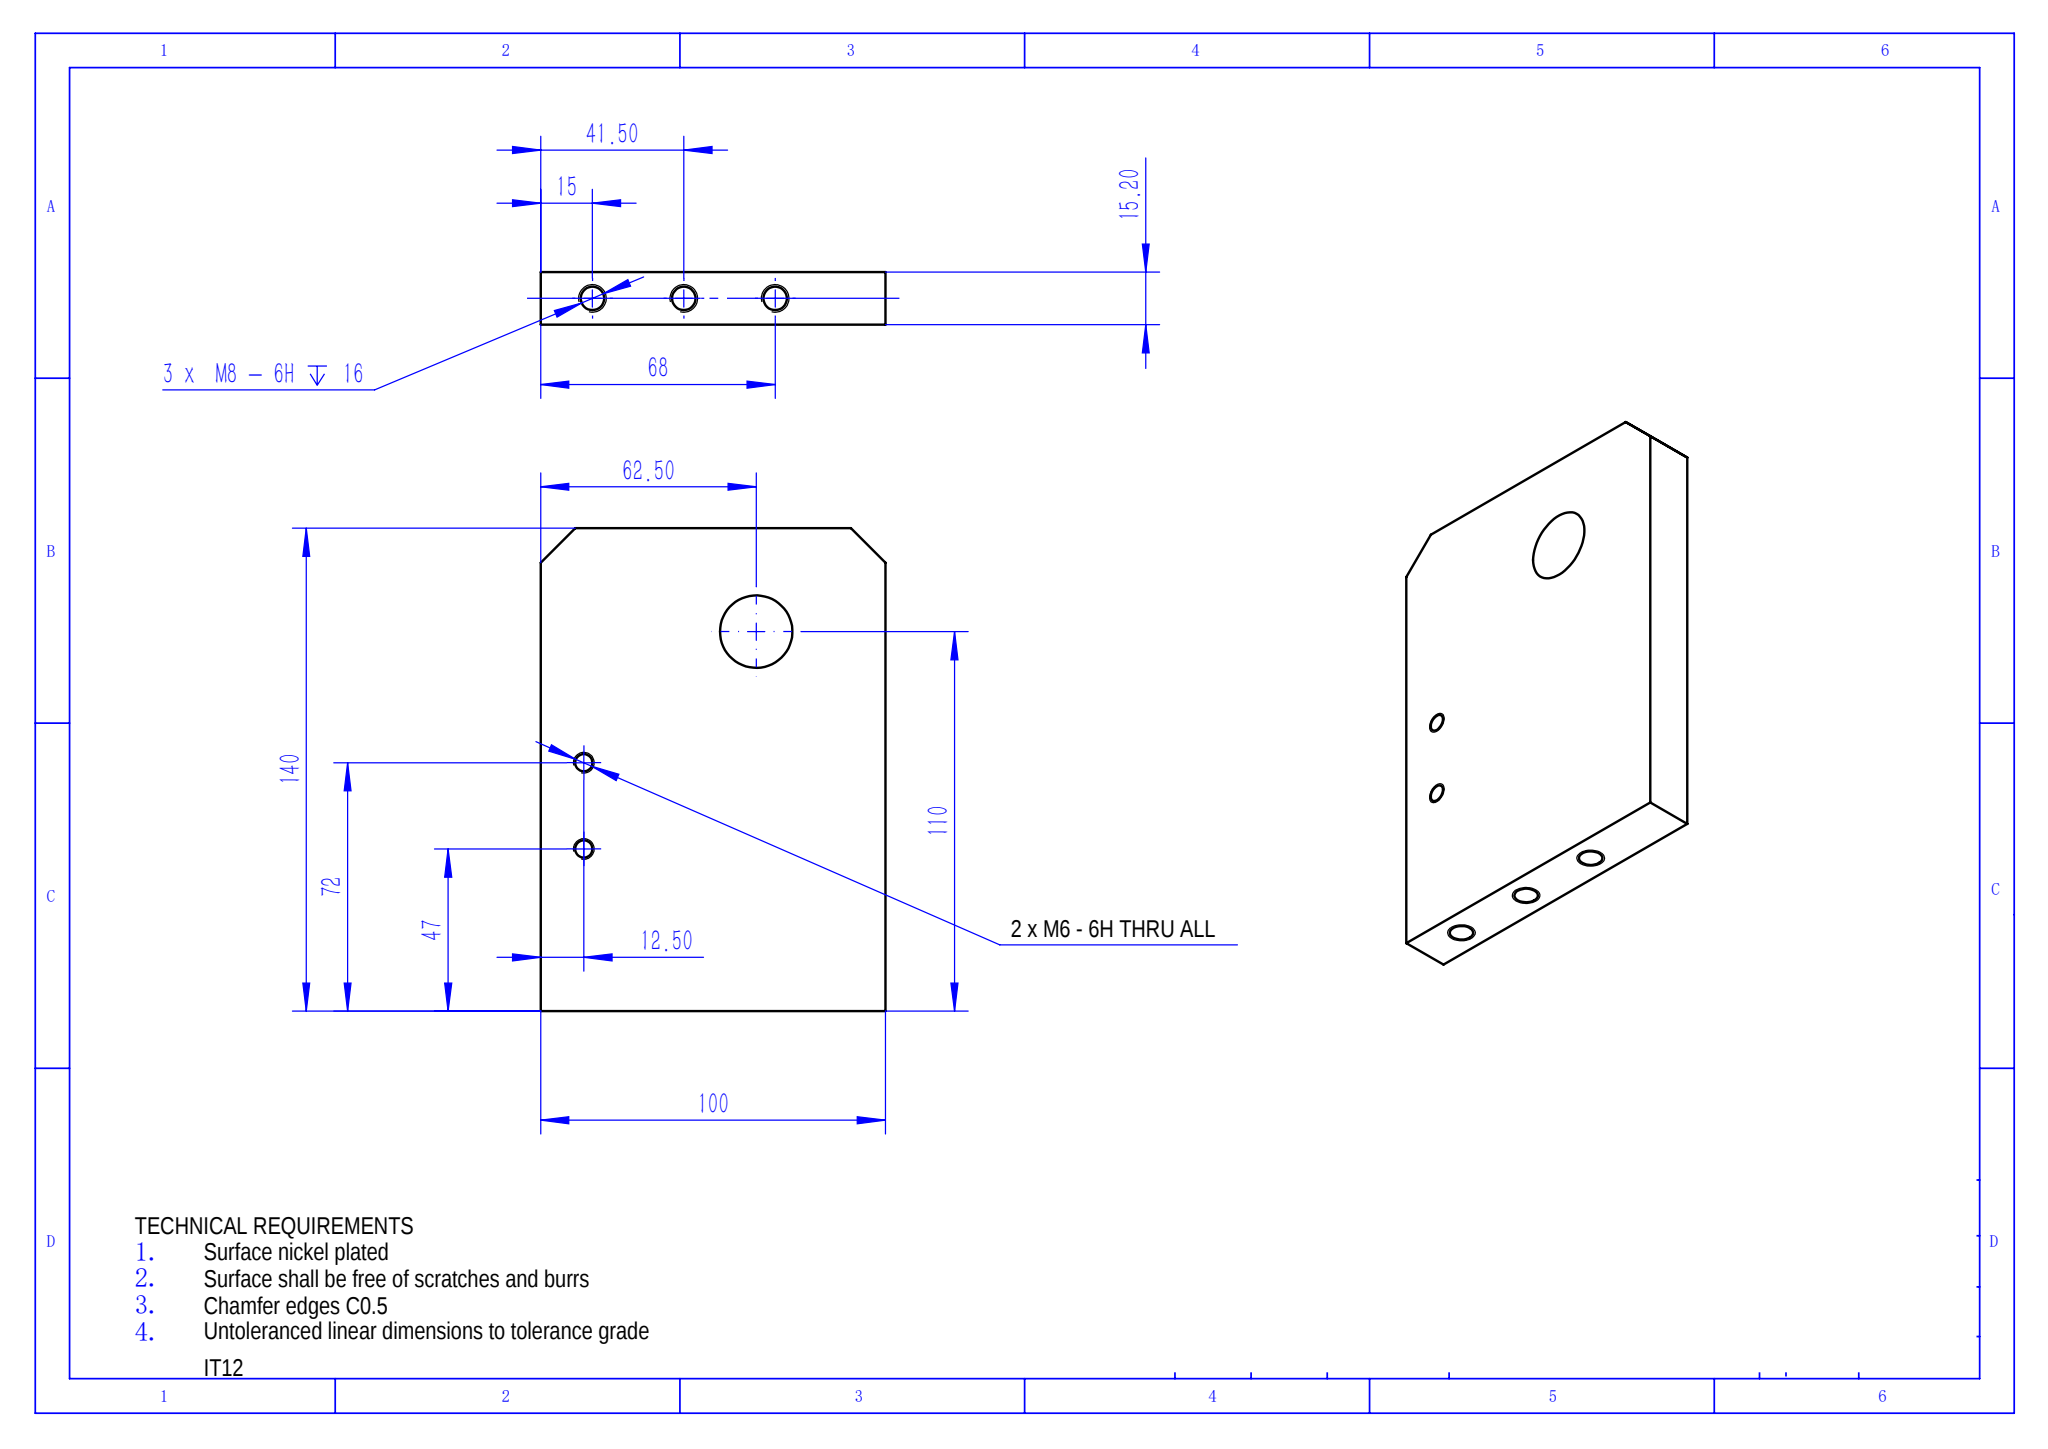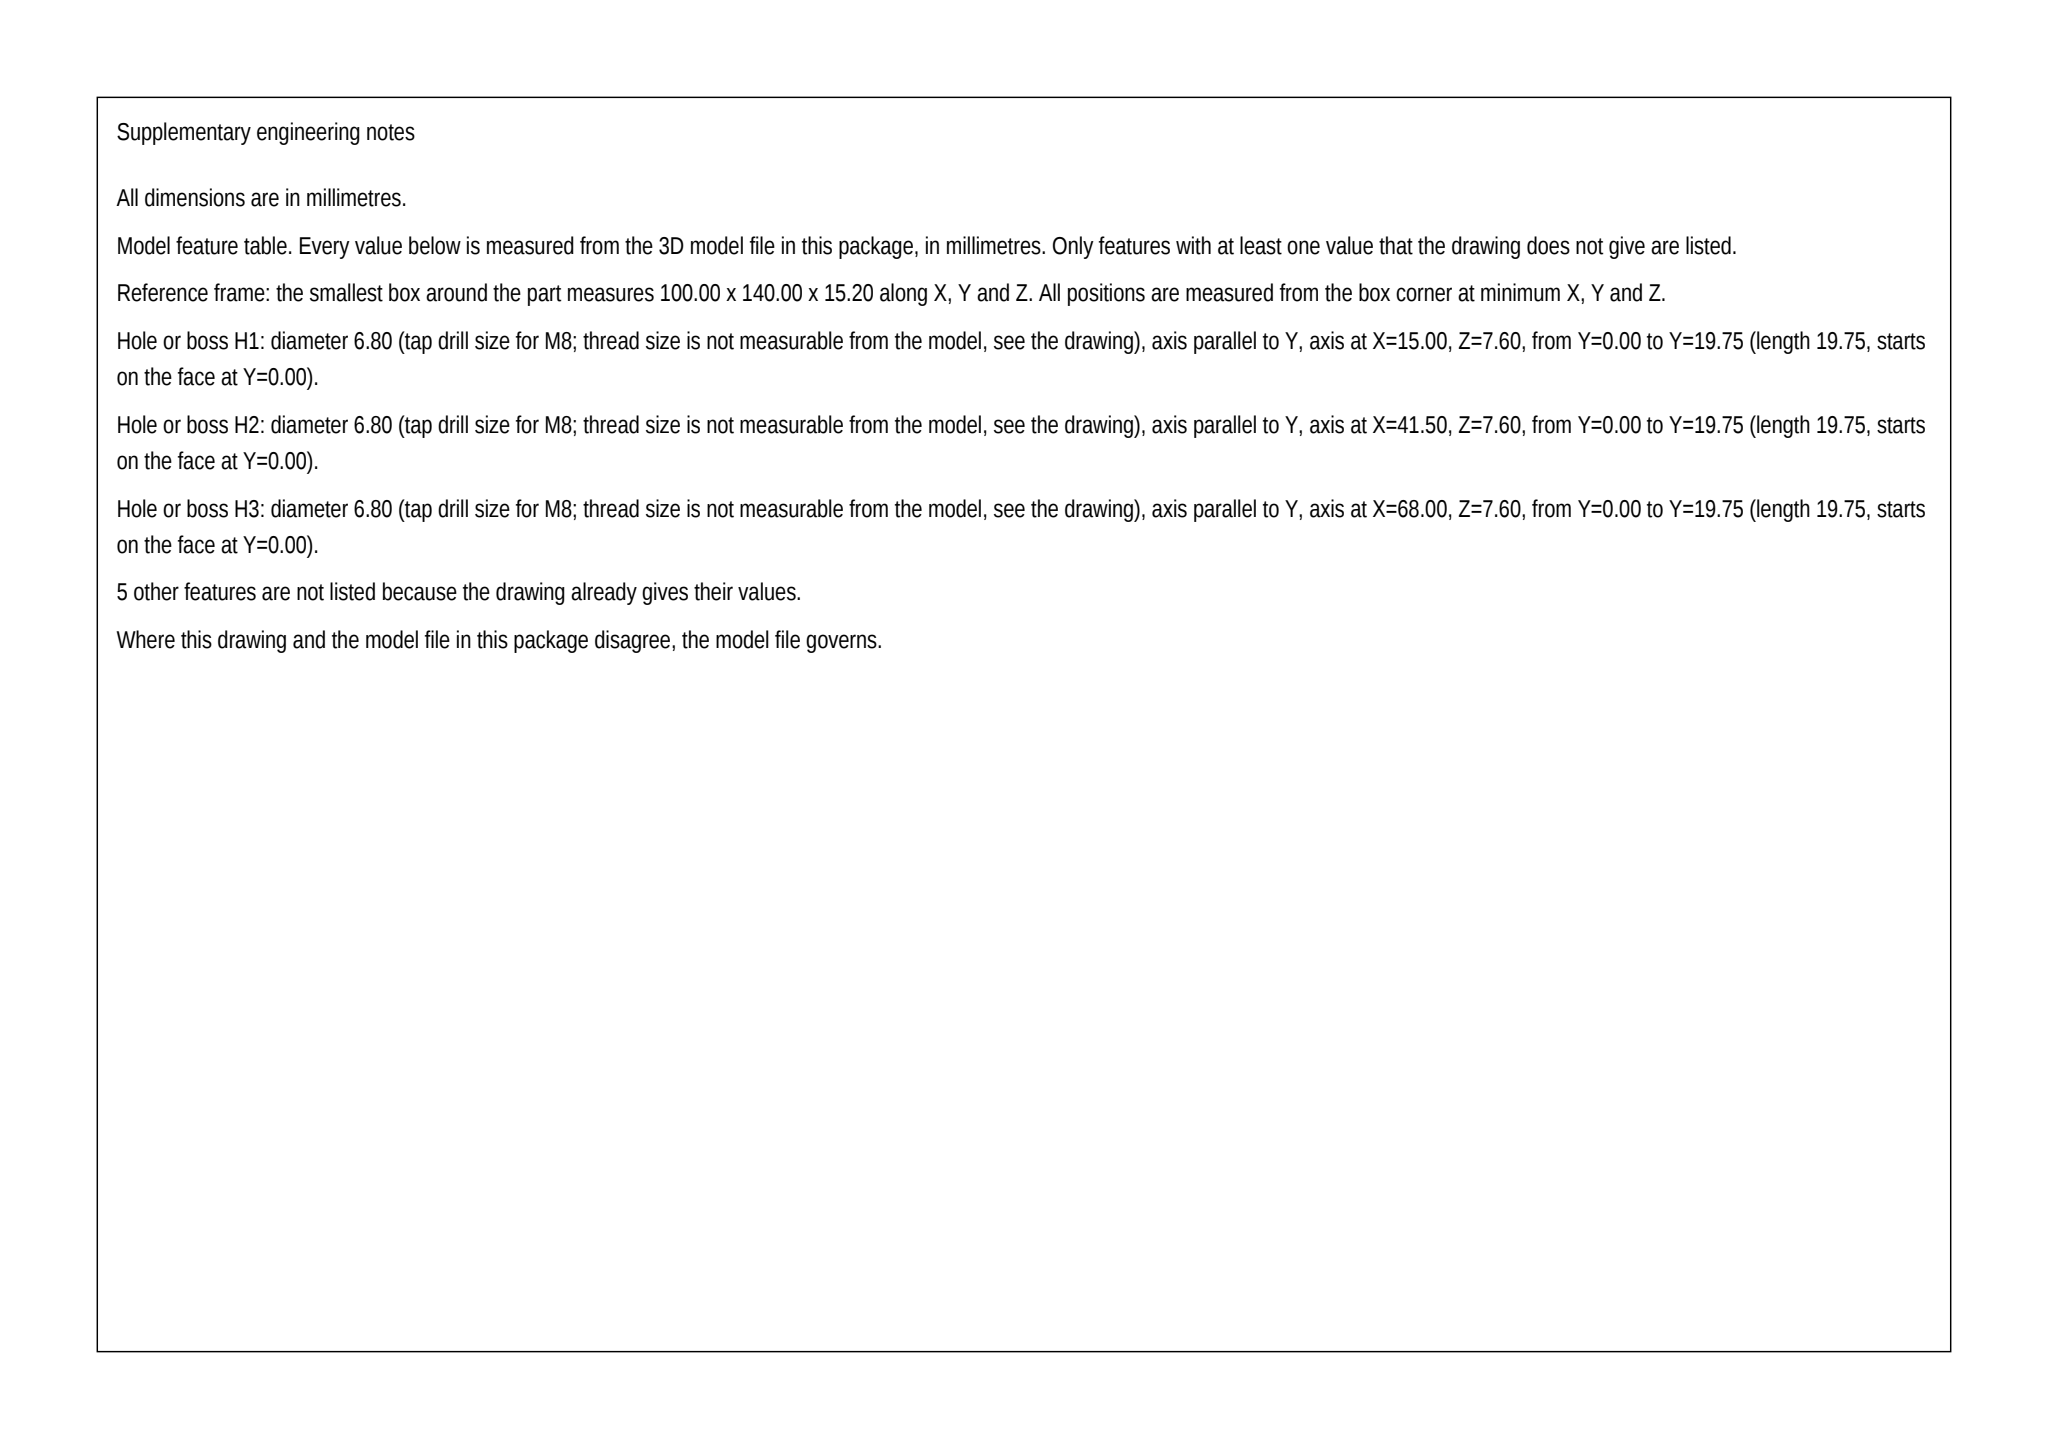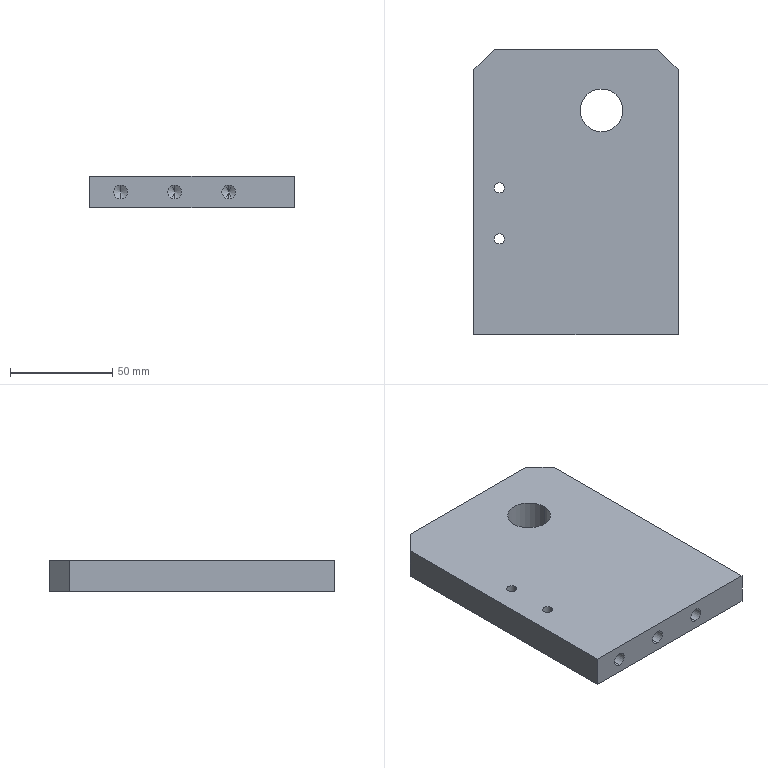Part | SolidWorks | mm | 1 solid | 26 faces | box 100 x 140 x 15.2 mm | volume 203192 mm3 | cylinder 12 | plane 8 | cone 6 | commonest cylinder face diameters 6.8 x6 5 x4 21 x2
Drawing notes:
FRONT VIEW: 2X C10 CHAMFER AT TOP CORNERS | from the solid: 100x140x15.2 plate, two cut corners on top edge of 140 face; chamfer legs 10
1X Ø21 THRU, 62.50 FROM LH EDGE, 110 FROM BOTTOM EDGE | from the solid: cylinder dia 21.0, axis z, pos (62.5,110.0), length 15.2 = full thickness
build123d program:
from build123d import *

# Parameters (mm, degrees)
SKETCH1_W             = 100
SKETCH1_H             = 140
BOSS_EXTRUDE1_DEPTH   = 15.2
SKETCH4_R             = 10.5
CUT_EXTRUDE1_DEPTH    = 173.717
CHAMFER1_SIZE         = 10
M8_TAPPED_HOLE2_D     = 6.8
M8_TAPPED_HOLE2_DEPTH = 19.75
M8_TAPPED_HOLE2_TIP   = 2.043
M6_TAPPED_HOLE2_D     = 5


with BuildPart() as part:
    # Sketch1 → Boss-Extrude1 (new body)
    with BuildSketch(Plane.XY):
        with Locations((50, 70)):
            Rectangle(SKETCH1_W, SKETCH1_H)
    extrude(amount=BOSS_EXTRUDE1_DEPTH)

    # Sketch4 → Cut-Extrude1 (cut, through all)
    with BuildSketch(Plane(origin=(0, 0, 0), x_dir=(-1, 0, 0), z_dir=(0, 0, -1))):
        with Locations((-62.5, 110)):
            Circle(SKETCH4_R)
    extrude(amount=-CUT_EXTRUDE1_DEPTH, mode=Mode.SUBTRACT)

    # Chamfer1
    chamfer1_edges = [part.edges().sort_by_distance(p)[0] for p in [
        (0, 140, 7.6),
        (100, 140, 7.6),
    ]]
    chamfer(chamfer1_edges, length=CHAMFER1_SIZE)

    # M8 Tapped Hole2
    with Locations(Plane(origin=(0, 0, 0), x_dir=(-1, 0, 0), z_dir=(0, -1, 0))):
        with Locations((-15, -7.6), (-41.5, -7.6), (-68, -7.6)):
            Hole(M8_TAPPED_HOLE2_D / 2, depth=M8_TAPPED_HOLE2_DEPTH)
            with Locations((0, 0, -(M8_TAPPED_HOLE2_DEPTH + M8_TAPPED_HOLE2_TIP / 2))):  # 118° drill point
                Cone(0, M8_TAPPED_HOLE2_D / 2, M8_TAPPED_HOLE2_TIP, mode=Mode.SUBTRACT)

    # M6 Tapped Hole2 (through all)
    with Locations(Plane.XY.offset(15.2)):
        with Locations((12.5, 72), (12.5, 47)):
            Hole(M6_TAPPED_HOLE2_D / 2)


solid = part.part
STEP:
#1=CARTESIAN_POINT('',(10.,72.,0.));
#2=VERTEX_POINT('',#1);
#3=CARTESIAN_POINT('',(15.,72.,0.));
#4=VERTEX_POINT('',#3);
#5=CARTESIAN_POINT('',(12.5,72.,0.));
#6=DIRECTION('',(0.,0.,1.));
#7=DIRECTION('',(1.,0.,0.));
#8=AXIS2_PLACEMENT_3D('',#5,#6,#7);
#9=CIRCLE('',#8,2.5);
#10=EDGE_CURVE('',#2,#4,#9,.T.);
#11=ORIENTED_EDGE('',*,*,#10,.F.);
#12=CARTESIAN_POINT('',(10.,72.,15.2));
#13=VERTEX_POINT('',#12);
#14=CARTESIAN_POINT('',(10.,72.,15.2));
#15=DIRECTION('',(0.,0.,1.));
#16=VECTOR('',#15,1000.);
#17=LINE('',#14,#16);
#18=EDGE_CURVE('',#2,#13,#17,.T.);
#19=ORIENTED_EDGE('',*,*,#18,.T.);
#20=CARTESIAN_POINT('',(15.,72.,15.2));
#21=VERTEX_POINT('',#20);
#22=CARTESIAN_POINT('',(12.5,72.,15.2));
#23=DIRECTION('',(0.,0.,1.));
#24=DIRECTION('',(1.,0.,0.));
#25=AXIS2_PLACEMENT_3D('',#22,#23,#24);
#26=CIRCLE('',#25,2.5);
#27=EDGE_CURVE('',#13,#21,#26,.T.);
#28=ORIENTED_EDGE('',*,*,#27,.T.);
#29=CARTESIAN_POINT('',(15.,72.,15.2));
#30=DIRECTION('',(0.,0.,1.));
#31=VECTOR('',#30,1000.);
#32=LINE('',#29,#31);
#33=EDGE_CURVE('',#4,#21,#32,.T.);
#34=ORIENTED_EDGE('',*,*,#33,.F.);
#35=EDGE_LOOP('',(#11,#19,#28,#34));
#36=FACE_OUTER_BOUND('',#35,.T.);
#37=CARTESIAN_POINT('',(12.5,72.,15.2));
#38=DIRECTION('',(0.,0.,1.));
#39=DIRECTION('',(1.,0.,0.));
#40=AXIS2_PLACEMENT_3D('',#37,#38,#39);
#41=CYLINDRICAL_SURFACE('',#40,2.5);
#42=ADVANCED_FACE('',(#36),#41,.F.);
#43=CARTESIAN_POINT('',(10.,47.,0.));
#44=VERTEX_POINT('',#43);
#45=CARTESIAN_POINT('',(15.,47.,0.));
#46=VERTEX_POINT('',#45);
#47=CARTESIAN_POINT('',(12.5,47.,0.));
#48=DIRECTION('',(0.,0.,1.));
#49=DIRECTION('',(1.,0.,0.));
#50=AXIS2_PLACEMENT_3D('',#47,#48,#49);
#51=CIRCLE('',#50,2.5);
#52=EDGE_CURVE('',#44,#46,#51,.T.);
#53=ORIENTED_EDGE('',*,*,#52,.F.);
#54=CARTESIAN_POINT('',(10.,47.,15.2));
#55=VERTEX_POINT('',#54);
#56=CARTESIAN_POINT('',(10.,47.,15.2));
#57=DIRECTION('',(0.,0.,1.));
#58=VECTOR('',#57,1000.);
#59=LINE('',#56,#58);
#60=EDGE_CURVE('',#44,#55,#59,.T.);
#61=ORIENTED_EDGE('',*,*,#60,.T.);
#62=CARTESIAN_POINT('',(15.,47.,15.2));
#63=VERTEX_POINT('',#62);
#64=CARTESIAN_POINT('',(12.5,47.,15.2));
#65=DIRECTION('',(0.,0.,1.));
#66=DIRECTION('',(1.,0.,0.));
#67=AXIS2_PLACEMENT_3D('',#64,#65,#66);
#68=CIRCLE('',#67,2.5);
#69=EDGE_CURVE('',#55,#63,#68,.T.);
#70=ORIENTED_EDGE('',*,*,#69,.T.);
#71=CARTESIAN_POINT('',(15.,47.,15.2));
#72=DIRECTION('',(0.,0.,1.));
#73=VECTOR('',#72,1000.);
#74=LINE('',#71,#73);
#75=EDGE_CURVE('',#46,#63,#74,.T.);
#76=ORIENTED_EDGE('',*,*,#75,.F.);
#77=EDGE_LOOP('',(#53,#61,#70,#76));
#78=FACE_OUTER_BOUND('',#77,.T.);
#79=CARTESIAN_POINT('',(12.5,47.,15.2));
#80=DIRECTION('',(0.,0.,1.));
#81=DIRECTION('',(1.,0.,0.));
#82=AXIS2_PLACEMENT_3D('',#79,#80,#81);
#83=CYLINDRICAL_SURFACE('',#82,2.5);
#84=ADVANCED_FACE('',(#78),#83,.F.);
#85=CARTESIAN_POINT('',(15.,19.75,11.));
#86=VERTEX_POINT('',#85);
#87=CARTESIAN_POINT('',(15.,19.75,4.2));
#88=VERTEX_POINT('',#87);
#89=CARTESIAN_POINT('',(15.,19.75,7.6));
#90=DIRECTION('',(0.,-1.,0.));
#91=DIRECTION('',(0.,0.,-1.));
#92=AXIS2_PLACEMENT_3D('',#89,#90,#91);
#93=CIRCLE('',#92,3.4);
#94=EDGE_CURVE('',#86,#88,#93,.T.);
#95=ORIENTED_EDGE('',*,*,#94,.F.);
#96=CARTESIAN_POINT('',(15.,-0.,11.));
#97=VERTEX_POINT('',#96);
#98=CARTESIAN_POINT('',(15.,0.,11.));
#99=DIRECTION('',(0.,-1.,0.));
#100=VECTOR('',#99,1000.);
#101=LINE('',#98,#100);
#102=EDGE_CURVE('',#86,#97,#101,.T.);
#103=ORIENTED_EDGE('',*,*,#102,.T.);
#104=CARTESIAN_POINT('',(15.,-0.,4.2));
#105=VERTEX_POINT('',#104);
#106=CARTESIAN_POINT('',(15.,-0.,7.6));
#107=DIRECTION('',(0.,-1.,0.));
#108=DIRECTION('',(0.,0.,-1.));
#109=AXIS2_PLACEMENT_3D('',#106,#107,#108);
#110=CIRCLE('',#109,3.4);
#111=EDGE_CURVE('',#97,#105,#110,.T.);
#112=ORIENTED_EDGE('',*,*,#111,.T.);
#113=CARTESIAN_POINT('',(15.,0.,4.2));
#114=DIRECTION('',(0.,-1.,0.));
#115=VECTOR('',#114,1000.);
#116=LINE('',#113,#115);
#117=EDGE_CURVE('',#88,#105,#116,.T.);
#118=ORIENTED_EDGE('',*,*,#117,.F.);
#119=EDGE_LOOP('',(#95,#103,#112,#118));
#120=FACE_OUTER_BOUND('',#119,.T.);
#121=CARTESIAN_POINT('',(15.,0.,7.6));
#122=DIRECTION('',(0.,-1.,0.));
#123=DIRECTION('',(0.,0.,-1.));
#124=AXIS2_PLACEMENT_3D('',#121,#122,#123);
#125=CYLINDRICAL_SURFACE('',#124,3.4);
#126=ADVANCED_FACE('',(#120),#125,.F.);
#127=CARTESIAN_POINT('',(15.,21.793,7.6));
#128=VERTEX_POINT('',#127);
#129=CARTESIAN_POINT('',(15.,19.75,4.2));
#130=DIRECTION('',(0.,-0.515,-0.8572));
#131=VECTOR('',#130,1000.);
#132=LINE('',#129,#131);
#133=EDGE_CURVE('',#128,#88,#132,.T.);
#134=ORIENTED_EDGE('',*,*,#133,.F.);
#135=CARTESIAN_POINT('',(15.,19.75,11.));
#136=DIRECTION('',(0.,-0.515,0.8572));
#137=VECTOR('',#136,1000.);
#138=LINE('',#135,#137);
#139=EDGE_CURVE('',#128,#86,#138,.T.);
#140=ORIENTED_EDGE('',*,*,#139,.T.);
#141=ORIENTED_EDGE('',*,*,#94,.T.);
#142=EDGE_LOOP('',(#134,#140,#141));
#143=FACE_OUTER_BOUND('',#142,.T.);
#144=CARTESIAN_POINT('',(15.,19.75,7.6));
#145=DIRECTION('',(0.,-1.,0.));
#146=DIRECTION('',(0.,0.,-1.));
#147=AXIS2_PLACEMENT_3D('',#144,#145,#146);
#148=CONICAL_SURFACE('',#147,3.4,1.03);
#149=ADVANCED_FACE('',(#143),#148,.F.);
#150=CARTESIAN_POINT('',(41.5,19.75,11.));
#151=VERTEX_POINT('',#150);
#152=CARTESIAN_POINT('',(41.5,19.75,4.2));
#153=VERTEX_POINT('',#152);
#154=CARTESIAN_POINT('',(41.5,19.75,7.6));
#155=DIRECTION('',(0.,-1.,0.));
#156=DIRECTION('',(0.,0.,-1.));
#157=AXIS2_PLACEMENT_3D('',#154,#155,#156);
#158=CIRCLE('',#157,3.4);
#159=EDGE_CURVE('',#151,#153,#158,.T.);
#160=ORIENTED_EDGE('',*,*,#159,.F.);
#161=CARTESIAN_POINT('',(41.5,-0.,11.));
#162=VERTEX_POINT('',#161);
#163=CARTESIAN_POINT('',(41.5,0.,11.));
#164=DIRECTION('',(0.,-1.,0.));
#165=VECTOR('',#164,1000.);
#166=LINE('',#163,#165);
#167=EDGE_CURVE('',#151,#162,#166,.T.);
#168=ORIENTED_EDGE('',*,*,#167,.T.);
#169=CARTESIAN_POINT('',(41.5,-0.,4.2));
#170=VERTEX_POINT('',#169);
#171=CARTESIAN_POINT('',(41.5,-0.,7.6));
#172=DIRECTION('',(0.,-1.,0.));
#173=DIRECTION('',(0.,0.,-1.));
#174=AXIS2_PLACEMENT_3D('',#171,#172,#173);
#175=CIRCLE('',#174,3.4);
#176=EDGE_CURVE('',#162,#170,#175,.T.);
#177=ORIENTED_EDGE('',*,*,#176,.T.);
#178=CARTESIAN_POINT('',(41.5,0.,4.2));
#179=DIRECTION('',(0.,-1.,0.));
#180=VECTOR('',#179,1000.);
#181=LINE('',#178,#180);
#182=EDGE_CURVE('',#153,#170,#181,.T.);
#183=ORIENTED_EDGE('',*,*,#182,.F.);
#184=EDGE_LOOP('',(#160,#168,#177,#183));
#185=FACE_OUTER_BOUND('',#184,.T.);
#186=CARTESIAN_POINT('',(41.5,0.,7.6));
#187=DIRECTION('',(0.,-1.,0.));
#188=DIRECTION('',(0.,0.,-1.));
#189=AXIS2_PLACEMENT_3D('',#186,#187,#188);
#190=CYLINDRICAL_SURFACE('',#189,3.4);
#191=ADVANCED_FACE('',(#185),#190,.F.);
#192=CARTESIAN_POINT('',(41.5,21.793,7.6));
#193=VERTEX_POINT('',#192);
#194=CARTESIAN_POINT('',(41.5,19.75,4.2));
#195=DIRECTION('',(0.,-0.515,-0.8572));
#196=VECTOR('',#195,1000.);
#197=LINE('',#194,#196);
#198=EDGE_CURVE('',#193,#153,#197,.T.);
#199=ORIENTED_EDGE('',*,*,#198,.F.);
#200=CARTESIAN_POINT('',(41.5,19.75,11.));
#201=DIRECTION('',(0.,-0.515,0.8572));
#202=VECTOR('',#201,1000.);
#203=LINE('',#200,#202);
#204=EDGE_CURVE('',#193,#151,#203,.T.);
#205=ORIENTED_EDGE('',*,*,#204,.T.);
#206=ORIENTED_EDGE('',*,*,#159,.T.);
#207=EDGE_LOOP('',(#199,#205,#206));
#208=FACE_OUTER_BOUND('',#207,.T.);
#209=CARTESIAN_POINT('',(41.5,19.75,7.6));
#210=DIRECTION('',(0.,-1.,0.));
#211=DIRECTION('',(0.,0.,-1.));
#212=AXIS2_PLACEMENT_3D('',#209,#210,#211);
#213=CONICAL_SURFACE('',#212,3.4,1.03);
#214=ADVANCED_FACE('',(#208),#213,.F.);
#215=CARTESIAN_POINT('',(68.,19.75,11.));
#216=VERTEX_POINT('',#215);
#217=CARTESIAN_POINT('',(68.,19.75,4.2));
#218=VERTEX_POINT('',#217);
#219=CARTESIAN_POINT('',(68.,19.75,7.6));
#220=DIRECTION('',(0.,-1.,0.));
#221=DIRECTION('',(0.,0.,-1.));
#222=AXIS2_PLACEMENT_3D('',#219,#220,#221);
#223=CIRCLE('',#222,3.4);
#224=EDGE_CURVE('',#216,#218,#223,.T.);
#225=ORIENTED_EDGE('',*,*,#224,.F.);
#226=CARTESIAN_POINT('',(68.,-0.,11.));
#227=VERTEX_POINT('',#226);
#228=CARTESIAN_POINT('',(68.,0.,11.));
#229=DIRECTION('',(0.,-1.,0.));
#230=VECTOR('',#229,1000.);
#231=LINE('',#228,#230);
#232=EDGE_CURVE('',#216,#227,#231,.T.);
#233=ORIENTED_EDGE('',*,*,#232,.T.);
#234=CARTESIAN_POINT('',(68.,-0.,4.2));
#235=VERTEX_POINT('',#234);
#236=CARTESIAN_POINT('',(68.,-0.,7.6));
#237=DIRECTION('',(0.,-1.,0.));
#238=DIRECTION('',(0.,0.,-1.));
#239=AXIS2_PLACEMENT_3D('',#236,#237,#238);
#240=CIRCLE('',#239,3.4);
#241=EDGE_CURVE('',#227,#235,#240,.T.);
#242=ORIENTED_EDGE('',*,*,#241,.T.);
#243=CARTESIAN_POINT('',(68.,0.,4.2));
#244=DIRECTION('',(0.,-1.,0.));
#245=VECTOR('',#244,1000.);
#246=LINE('',#243,#245);
#247=EDGE_CURVE('',#218,#235,#246,.T.);
#248=ORIENTED_EDGE('',*,*,#247,.F.);
#249=EDGE_LOOP('',(#225,#233,#242,#248));
#250=FACE_OUTER_BOUND('',#249,.T.);
#251=CARTESIAN_POINT('',(68.,0.,7.6));
#252=DIRECTION('',(0.,-1.,0.));
#253=DIRECTION('',(0.,0.,-1.));
#254=AXIS2_PLACEMENT_3D('',#251,#252,#253);
#255=CYLINDRICAL_SURFACE('',#254,3.4);
#256=ADVANCED_FACE('',(#250),#255,.F.);
#257=CARTESIAN_POINT('',(68.,21.793,7.6));
#258=VERTEX_POINT('',#257);
#259=CARTESIAN_POINT('',(68.,19.75,4.2));
#260=DIRECTION('',(0.,-0.515,-0.8572));
#261=VECTOR('',#260,1000.);
#262=LINE('',#259,#261);
#263=EDGE_CURVE('',#258,#218,#262,.T.);
#264=ORIENTED_EDGE('',*,*,#263,.F.);
#265=CARTESIAN_POINT('',(68.,19.75,11.));
#266=DIRECTION('',(0.,-0.515,0.8572));
#267=VECTOR('',#266,1000.);
#268=LINE('',#265,#267);
#269=EDGE_CURVE('',#258,#216,#268,.T.);
#270=ORIENTED_EDGE('',*,*,#269,.T.);
#271=ORIENTED_EDGE('',*,*,#224,.T.);
#272=EDGE_LOOP('',(#264,#270,#271));
#273=FACE_OUTER_BOUND('',#272,.T.);
#274=CARTESIAN_POINT('',(68.,19.75,7.6));
#275=DIRECTION('',(0.,-1.,0.));
#276=DIRECTION('',(0.,0.,-1.));
#277=AXIS2_PLACEMENT_3D('',#274,#275,#276);
#278=CONICAL_SURFACE('',#277,3.4,1.03);
#279=ADVANCED_FACE('',(#273),#278,.F.);
#280=CARTESIAN_POINT('',(73.,110.,15.2));
#281=VERTEX_POINT('',#280);
#282=CARTESIAN_POINT('',(52.,110.,15.2));
#283=VERTEX_POINT('',#282);
#284=CARTESIAN_POINT('',(62.5,110.,15.2));
#285=DIRECTION('',(0.,0.,-1.));
#286=DIRECTION('',(-1.,0.,0.));
#287=AXIS2_PLACEMENT_3D('',#284,#285,#286);
#288=CIRCLE('',#287,10.5);
#289=EDGE_CURVE('',#281,#283,#288,.T.);
#290=ORIENTED_EDGE('',*,*,#289,.F.);
#291=CARTESIAN_POINT('',(73.,110.,0.));
#292=VERTEX_POINT('',#291);
#293=CARTESIAN_POINT('',(73.,110.,15.2));
#294=DIRECTION('',(0.,0.,-1.));
#295=VECTOR('',#294,1000.);
#296=LINE('',#293,#295);
#297=EDGE_CURVE('',#281,#292,#296,.T.);
#298=ORIENTED_EDGE('',*,*,#297,.T.);
#299=CARTESIAN_POINT('',(52.,110.,0.));
#300=VERTEX_POINT('',#299);
#301=CARTESIAN_POINT('',(62.5,110.,0.));
#302=DIRECTION('',(0.,0.,-1.));
#303=DIRECTION('',(-1.,0.,0.));
#304=AXIS2_PLACEMENT_3D('',#301,#302,#303);
#305=CIRCLE('',#304,10.5);
#306=EDGE_CURVE('',#292,#300,#305,.T.);
#307=ORIENTED_EDGE('',*,*,#306,.T.);
#308=CARTESIAN_POINT('',(52.,110.,15.2));
#309=DIRECTION('',(0.,0.,-1.));
#310=VECTOR('',#309,1000.);
#311=LINE('',#308,#310);
#312=EDGE_CURVE('',#283,#300,#311,.T.);
#313=ORIENTED_EDGE('',*,*,#312,.F.);
#314=EDGE_LOOP('',(#290,#298,#307,#313));
#315=FACE_OUTER_BOUND('',#314,.T.);
#316=CARTESIAN_POINT('',(62.5,110.,15.2));
#317=DIRECTION('',(0.,0.,-1.));
#318=DIRECTION('',(-1.,0.,0.));
#319=AXIS2_PLACEMENT_3D('',#316,#317,#318);
#320=CYLINDRICAL_SURFACE('',#319,10.5);
#321=ADVANCED_FACE('',(#315),#320,.F.);
#322=CARTESIAN_POINT('',(90.,140.,0.));
#323=VERTEX_POINT('',#322);
#324=CARTESIAN_POINT('',(10.,140.,0.));
#325=VERTEX_POINT('',#324);
#326=CARTESIAN_POINT('',(0.,140.,0.));
#327=DIRECTION('',(-1.,0.,0.));
#328=VECTOR('',#327,1000.);
#329=LINE('',#326,#328);
#330=EDGE_CURVE('',#323,#325,#329,.T.);
#331=ORIENTED_EDGE('',*,*,#330,.F.);
#332=CARTESIAN_POINT('',(100.,130.,0.));
#333=VERTEX_POINT('',#332);
#334=CARTESIAN_POINT('',(115.,115.,0.));
#335=DIRECTION('',(0.7071,-0.7071,0.));
#336=VECTOR('',#335,1000.);
#337=LINE('',#334,#336);
#338=EDGE_CURVE('',#323,#333,#337,.T.);
#339=ORIENTED_EDGE('',*,*,#338,.T.);
#340=CARTESIAN_POINT('',(100.,0.,0.));
#341=VERTEX_POINT('',#340);
#342=CARTESIAN_POINT('',(100.,0.,0.));
#343=DIRECTION('',(0.,1.,0.));
#344=VECTOR('',#343,1000.);
#345=LINE('',#342,#344);
#346=EDGE_CURVE('',#341,#333,#345,.T.);
#347=ORIENTED_EDGE('',*,*,#346,.F.);
#348=CARTESIAN_POINT('',(0.,0.,0.));
#349=VERTEX_POINT('',#348);
#350=CARTESIAN_POINT('',(0.,0.,0.));
#351=DIRECTION('',(1.,0.,0.));
#352=VECTOR('',#351,1000.);
#353=LINE('',#350,#352);
#354=EDGE_CURVE('',#349,#341,#353,.T.);
#355=ORIENTED_EDGE('',*,*,#354,.F.);
#356=CARTESIAN_POINT('',(0.,130.,0.));
#357=VERTEX_POINT('',#356);
#358=CARTESIAN_POINT('',(0.,0.,0.));
#359=DIRECTION('',(0.,-1.,0.));
#360=VECTOR('',#359,1000.);
#361=LINE('',#358,#360);
#362=EDGE_CURVE('',#357,#349,#361,.T.);
#363=ORIENTED_EDGE('',*,*,#362,.F.);
#364=CARTESIAN_POINT('',(-65.,65.,0.));
#365=DIRECTION('',(0.7071,0.7071,0.));
#366=VECTOR('',#365,1000.);
#367=LINE('',#364,#366);
#368=EDGE_CURVE('',#357,#325,#367,.T.);
#369=ORIENTED_EDGE('',*,*,#368,.T.);
#370=EDGE_LOOP('',(#331,#339,#347,#355,#363,#369));
#371=FACE_OUTER_BOUND('',#370,.T.);
#372=CARTESIAN_POINT('',(62.5,110.,0.));
#373=DIRECTION('',(0.,0.,-1.));
#374=DIRECTION('',(-1.,0.,0.));
#375=AXIS2_PLACEMENT_3D('',#372,#373,#374);
#376=CIRCLE('',#375,10.5);
#377=EDGE_CURVE('',#300,#292,#376,.T.);
#378=ORIENTED_EDGE('',*,*,#377,.F.);
#379=ORIENTED_EDGE('',*,*,#306,.F.);
#380=EDGE_LOOP('',(#378,#379));
#381=FACE_BOUND('',#380,.T.);
#382=CARTESIAN_POINT('',(12.5,47.,0.));
#383=DIRECTION('',(0.,0.,1.));
#384=DIRECTION('',(1.,0.,0.));
#385=AXIS2_PLACEMENT_3D('',#382,#383,#384);
#386=CIRCLE('',#385,2.5);
#387=EDGE_CURVE('',#46,#44,#386,.T.);
#388=ORIENTED_EDGE('',*,*,#387,.T.);
#389=ORIENTED_EDGE('',*,*,#52,.T.);
#390=EDGE_LOOP('',(#388,#389));
#391=FACE_BOUND('',#390,.T.);
#392=CARTESIAN_POINT('',(12.5,72.,0.));
#393=DIRECTION('',(0.,0.,1.));
#394=DIRECTION('',(1.,0.,0.));
#395=AXIS2_PLACEMENT_3D('',#392,#393,#394);
#396=CIRCLE('',#395,2.5);
#397=EDGE_CURVE('',#4,#2,#396,.T.);
#398=ORIENTED_EDGE('',*,*,#397,.T.);
#399=ORIENTED_EDGE('',*,*,#10,.T.);
#400=EDGE_LOOP('',(#398,#399));
#401=FACE_BOUND('',#400,.T.);
#402=CARTESIAN_POINT('',(0.,0.,0.));
#403=DIRECTION('',(0.,0.,-1.));
#404=DIRECTION('',(-1.,0.,0.));
#405=AXIS2_PLACEMENT_3D('',#402,#403,#404);
#406=PLANE('',#405);
#407=ADVANCED_FACE('',(#371,#381,#391,#401),#406,.T.);
#408=CARTESIAN_POINT('',(0.,130.,15.2));
#409=VERTEX_POINT('',#408);
#410=CARTESIAN_POINT('',(0.,0.,15.2));
#411=VERTEX_POINT('',#410);
#412=CARTESIAN_POINT('',(0.,0.,15.2));
#413=DIRECTION('',(0.,-1.,0.));
#414=VECTOR('',#413,1000.);
#415=LINE('',#412,#414);
#416=EDGE_CURVE('',#409,#411,#415,.T.);
#417=ORIENTED_EDGE('',*,*,#416,.F.);
#418=CARTESIAN_POINT('',(0.,130.,15.2));
#419=DIRECTION('',(0.,0.,-1.));
#420=VECTOR('',#419,1000.);
#421=LINE('',#418,#420);
#422=EDGE_CURVE('',#409,#357,#421,.T.);
#423=ORIENTED_EDGE('',*,*,#422,.T.);
#424=ORIENTED_EDGE('',*,*,#362,.T.);
#425=CARTESIAN_POINT('',(0.,0.,15.2));
#426=DIRECTION('',(0.,0.,-1.));
#427=VECTOR('',#426,1000.);
#428=LINE('',#425,#427);
#429=EDGE_CURVE('',#411,#349,#428,.T.);
#430=ORIENTED_EDGE('',*,*,#429,.F.);
#431=EDGE_LOOP('',(#417,#423,#424,#430));
#432=FACE_OUTER_BOUND('',#431,.T.);
#433=CARTESIAN_POINT('',(0.,0.,15.2));
#434=DIRECTION('',(1.,0.,0.));
#435=DIRECTION('',(0.,0.,-1.));
#436=AXIS2_PLACEMENT_3D('',#433,#434,#435);
#437=PLANE('',#436);
#438=ADVANCED_FACE('',(#432),#437,.F.);
#439=CARTESIAN_POINT('',(15.,-0.,7.6));
#440=DIRECTION('',(0.,-1.,0.));
#441=DIRECTION('',(0.,0.,-1.));
#442=AXIS2_PLACEMENT_3D('',#439,#440,#441);
#443=CIRCLE('',#442,3.4);
#444=EDGE_CURVE('',#105,#97,#443,.T.);
#445=ORIENTED_EDGE('',*,*,#444,.F.);
#446=ORIENTED_EDGE('',*,*,#111,.F.);
#447=EDGE_LOOP('',(#445,#446));
#448=FACE_BOUND('',#447,.T.);
#449=CARTESIAN_POINT('',(41.5,-0.,7.6));
#450=DIRECTION('',(0.,-1.,0.));
#451=DIRECTION('',(0.,0.,-1.));
#452=AXIS2_PLACEMENT_3D('',#449,#450,#451);
#453=CIRCLE('',#452,3.4);
#454=EDGE_CURVE('',#170,#162,#453,.T.);
#455=ORIENTED_EDGE('',*,*,#454,.F.);
#456=ORIENTED_EDGE('',*,*,#176,.F.);
#457=EDGE_LOOP('',(#455,#456));
#458=FACE_BOUND('',#457,.T.);
#459=CARTESIAN_POINT('',(68.,-0.,7.6));
#460=DIRECTION('',(0.,-1.,0.));
#461=DIRECTION('',(0.,0.,-1.));
#462=AXIS2_PLACEMENT_3D('',#459,#460,#461);
#463=CIRCLE('',#462,3.4);
#464=EDGE_CURVE('',#235,#227,#463,.T.);
#465=ORIENTED_EDGE('',*,*,#464,.F.);
#466=ORIENTED_EDGE('',*,*,#241,.F.);
#467=EDGE_LOOP('',(#465,#466));
#468=FACE_BOUND('',#467,.T.);
#469=ORIENTED_EDGE('',*,*,#354,.T.);
#470=CARTESIAN_POINT('',(100.,0.,15.2));
#471=VERTEX_POINT('',#470);
#472=CARTESIAN_POINT('',(100.,0.,15.2));
#473=DIRECTION('',(0.,0.,-1.));
#474=VECTOR('',#473,1000.);
#475=LINE('',#472,#474);
#476=EDGE_CURVE('',#471,#341,#475,.T.);
#477=ORIENTED_EDGE('',*,*,#476,.F.);
#478=CARTESIAN_POINT('',(0.,0.,15.2));
#479=DIRECTION('',(1.,0.,0.));
#480=VECTOR('',#479,1000.);
#481=LINE('',#478,#480);
#482=EDGE_CURVE('',#411,#471,#481,.T.);
#483=ORIENTED_EDGE('',*,*,#482,.F.);
#484=ORIENTED_EDGE('',*,*,#429,.T.);
#485=EDGE_LOOP('',(#469,#477,#483,#484));
#486=FACE_OUTER_BOUND('',#485,.T.);
#487=CARTESIAN_POINT('',(0.,0.,15.2));
#488=DIRECTION('',(0.,1.,0.));
#489=DIRECTION('',(0.,0.,1.));
#490=AXIS2_PLACEMENT_3D('',#487,#488,#489);
#491=PLANE('',#490);
#492=ADVANCED_FACE('',(#448,#458,#468,#486),#491,.F.);
#493=ORIENTED_EDGE('',*,*,#346,.T.);
#494=CARTESIAN_POINT('',(100.,130.,15.2));
#495=VERTEX_POINT('',#494);
#496=CARTESIAN_POINT('',(100.,130.,15.2));
#497=DIRECTION('',(0.,0.,1.));
#498=VECTOR('',#497,1000.);
#499=LINE('',#496,#498);
#500=EDGE_CURVE('',#333,#495,#499,.T.);
#501=ORIENTED_EDGE('',*,*,#500,.T.);
#502=CARTESIAN_POINT('',(100.,0.,15.2));
#503=DIRECTION('',(0.,1.,0.));
#504=VECTOR('',#503,1000.);
#505=LINE('',#502,#504);
#506=EDGE_CURVE('',#471,#495,#505,.T.);
#507=ORIENTED_EDGE('',*,*,#506,.F.);
#508=ORIENTED_EDGE('',*,*,#476,.T.);
#509=EDGE_LOOP('',(#493,#501,#507,#508));
#510=FACE_OUTER_BOUND('',#509,.T.);
#511=CARTESIAN_POINT('',(100.,0.,15.2));
#512=DIRECTION('',(-1.,0.,0.));
#513=DIRECTION('',(0.,0.,1.));
#514=AXIS2_PLACEMENT_3D('',#511,#512,#513);
#515=PLANE('',#514);
#516=ADVANCED_FACE('',(#510),#515,.F.);
#517=CARTESIAN_POINT('',(90.,140.,15.2));
#518=VERTEX_POINT('',#517);
#519=CARTESIAN_POINT('',(10.,140.,15.2));
#520=VERTEX_POINT('',#519);
#521=CARTESIAN_POINT('',(0.,140.,15.2));
#522=DIRECTION('',(-1.,0.,0.));
#523=VECTOR('',#522,1000.);
#524=LINE('',#521,#523);
#525=EDGE_CURVE('',#518,#520,#524,.T.);
#526=ORIENTED_EDGE('',*,*,#525,.F.);
#527=CARTESIAN_POINT('',(90.,140.,15.2));
#528=DIRECTION('',(0.,0.,-1.));
#529=VECTOR('',#528,1000.);
#530=LINE('',#527,#529);
#531=EDGE_CURVE('',#518,#323,#530,.T.);
#532=ORIENTED_EDGE('',*,*,#531,.T.);
#533=ORIENTED_EDGE('',*,*,#330,.T.);
#534=CARTESIAN_POINT('',(10.,140.,15.2));
#535=DIRECTION('',(0.,0.,1.));
#536=VECTOR('',#535,1000.);
#537=LINE('',#534,#536);
#538=EDGE_CURVE('',#325,#520,#537,.T.);
#539=ORIENTED_EDGE('',*,*,#538,.T.);
#540=EDGE_LOOP('',(#526,#532,#533,#539));
#541=FACE_OUTER_BOUND('',#540,.T.);
#542=CARTESIAN_POINT('',(0.,140.,15.2));
#543=DIRECTION('',(0.,-1.,0.));
#544=DIRECTION('',(0.,0.,-1.));
#545=AXIS2_PLACEMENT_3D('',#542,#543,#544);
#546=PLANE('',#545);
#547=ADVANCED_FACE('',(#541),#546,.F.);
#548=CARTESIAN_POINT('',(12.5,72.,15.2));
#549=DIRECTION('',(0.,0.,1.));
#550=DIRECTION('',(1.,0.,0.));
#551=AXIS2_PLACEMENT_3D('',#548,#549,#550);
#552=CIRCLE('',#551,2.5);
#553=EDGE_CURVE('',#21,#13,#552,.T.);
#554=ORIENTED_EDGE('',*,*,#553,.F.);
#555=ORIENTED_EDGE('',*,*,#27,.F.);
#556=EDGE_LOOP('',(#554,#555));
#557=FACE_BOUND('',#556,.T.);
#558=CARTESIAN_POINT('',(12.5,47.,15.2));
#559=DIRECTION('',(0.,0.,1.));
#560=DIRECTION('',(1.,0.,0.));
#561=AXIS2_PLACEMENT_3D('',#558,#559,#560);
#562=CIRCLE('',#561,2.5);
#563=EDGE_CURVE('',#63,#55,#562,.T.);
#564=ORIENTED_EDGE('',*,*,#563,.F.);
#565=ORIENTED_EDGE('',*,*,#69,.F.);
#566=EDGE_LOOP('',(#564,#565));
#567=FACE_BOUND('',#566,.T.);
#568=CARTESIAN_POINT('',(62.5,110.,15.2));
#569=DIRECTION('',(0.,0.,-1.));
#570=DIRECTION('',(-1.,0.,0.));
#571=AXIS2_PLACEMENT_3D('',#568,#569,#570);
#572=CIRCLE('',#571,10.5);
#573=EDGE_CURVE('',#283,#281,#572,.T.);
#574=ORIENTED_EDGE('',*,*,#573,.T.);
#575=ORIENTED_EDGE('',*,*,#289,.T.);
#576=EDGE_LOOP('',(#574,#575));
#577=FACE_BOUND('',#576,.T.);
#578=ORIENTED_EDGE('',*,*,#506,.T.);
#579=CARTESIAN_POINT('',(90.,140.,15.2));
#580=DIRECTION('',(-0.7071,0.7071,0.));
#581=VECTOR('',#580,1000.);
#582=LINE('',#579,#581);
#583=EDGE_CURVE('',#495,#518,#582,.T.);
#584=ORIENTED_EDGE('',*,*,#583,.T.);
#585=ORIENTED_EDGE('',*,*,#525,.T.);
#586=CARTESIAN_POINT('',(0.,130.,15.2));
#587=DIRECTION('',(-0.7071,-0.7071,0.));
#588=VECTOR('',#587,1000.);
#589=LINE('',#586,#588);
#590=EDGE_CURVE('',#520,#409,#589,.T.);
#591=ORIENTED_EDGE('',*,*,#590,.T.);
#592=ORIENTED_EDGE('',*,*,#416,.T.);
#593=ORIENTED_EDGE('',*,*,#482,.T.);
#594=EDGE_LOOP('',(#578,#584,#585,#591,#592,#593));
#595=FACE_OUTER_BOUND('',#594,.T.);
#596=CARTESIAN_POINT('',(0.,0.,15.2));
#597=DIRECTION('',(0.,0.,-1.));
#598=DIRECTION('',(-1.,0.,0.));
#599=AXIS2_PLACEMENT_3D('',#596,#597,#598);
#600=PLANE('',#599);
#601=ADVANCED_FACE('',(#557,#567,#577,#595),#600,.F.);
#602=ORIENTED_EDGE('',*,*,#297,.F.);
#603=ORIENTED_EDGE('',*,*,#573,.F.);
#604=ORIENTED_EDGE('',*,*,#312,.T.);
#605=ORIENTED_EDGE('',*,*,#377,.T.);
#606=EDGE_LOOP('',(#602,#603,#604,#605));
#607=FACE_OUTER_BOUND('',#606,.T.);
#608=CARTESIAN_POINT('',(62.5,110.,15.2));
#609=DIRECTION('',(0.,0.,-1.));
#610=DIRECTION('',(-1.,0.,0.));
#611=AXIS2_PLACEMENT_3D('',#608,#609,#610);
#612=CYLINDRICAL_SURFACE('',#611,10.5);
#613=ADVANCED_FACE('',(#607),#612,.F.);
#614=ORIENTED_EDGE('',*,*,#583,.F.);
#615=ORIENTED_EDGE('',*,*,#500,.F.);
#616=ORIENTED_EDGE('',*,*,#338,.F.);
#617=ORIENTED_EDGE('',*,*,#531,.F.);
#618=EDGE_LOOP('',(#614,#615,#616,#617));
#619=FACE_OUTER_BOUND('',#618,.T.);
#620=CARTESIAN_POINT('',(90.,140.,15.2));
#621=DIRECTION('',(-0.7071,-0.7071,0.));
#622=DIRECTION('',(0.,0.,-1.));
#623=AXIS2_PLACEMENT_3D('',#620,#621,#622);
#624=PLANE('',#623);
#625=ADVANCED_FACE('',(#619),#624,.F.);
#626=ORIENTED_EDGE('',*,*,#590,.F.);
#627=ORIENTED_EDGE('',*,*,#538,.F.);
#628=ORIENTED_EDGE('',*,*,#368,.F.);
#629=ORIENTED_EDGE('',*,*,#422,.F.);
#630=EDGE_LOOP('',(#626,#627,#628,#629));
#631=FACE_OUTER_BOUND('',#630,.T.);
#632=CARTESIAN_POINT('',(0.,130.,15.2));
#633=DIRECTION('',(0.7071,-0.7071,0.));
#634=DIRECTION('',(0.,0.,-1.));
#635=AXIS2_PLACEMENT_3D('',#632,#633,#634);
#636=PLANE('',#635);
#637=ADVANCED_FACE('',(#631),#636,.F.);
#638=ORIENTED_EDGE('',*,*,#269,.F.);
#639=ORIENTED_EDGE('',*,*,#263,.T.);
#640=CARTESIAN_POINT('',(68.,19.75,7.6));
#641=DIRECTION('',(0.,-1.,0.));
#642=DIRECTION('',(0.,0.,-1.));
#643=AXIS2_PLACEMENT_3D('',#640,#641,#642);
#644=CIRCLE('',#643,3.4);
#645=EDGE_CURVE('',#218,#216,#644,.T.);
#646=ORIENTED_EDGE('',*,*,#645,.T.);
#647=EDGE_LOOP('',(#638,#639,#646));
#648=FACE_OUTER_BOUND('',#647,.T.);
#649=CARTESIAN_POINT('',(68.,19.75,7.6));
#650=DIRECTION('',(0.,-1.,0.));
#651=DIRECTION('',(0.,0.,-1.));
#652=AXIS2_PLACEMENT_3D('',#649,#650,#651);
#653=CONICAL_SURFACE('',#652,3.4,1.03);
#654=ADVANCED_FACE('',(#648),#653,.F.);
#655=ORIENTED_EDGE('',*,*,#232,.F.);
#656=ORIENTED_EDGE('',*,*,#645,.F.);
#657=ORIENTED_EDGE('',*,*,#247,.T.);
#658=ORIENTED_EDGE('',*,*,#464,.T.);
#659=EDGE_LOOP('',(#655,#656,#657,#658));
#660=FACE_OUTER_BOUND('',#659,.T.);
#661=CARTESIAN_POINT('',(68.,0.,7.6));
#662=DIRECTION('',(0.,-1.,0.));
#663=DIRECTION('',(0.,0.,-1.));
#664=AXIS2_PLACEMENT_3D('',#661,#662,#663);
#665=CYLINDRICAL_SURFACE('',#664,3.4);
#666=ADVANCED_FACE('',(#660),#665,.F.);
#667=ORIENTED_EDGE('',*,*,#204,.F.);
#668=ORIENTED_EDGE('',*,*,#198,.T.);
#669=CARTESIAN_POINT('',(41.5,19.75,7.6));
#670=DIRECTION('',(0.,-1.,0.));
#671=DIRECTION('',(0.,0.,-1.));
#672=AXIS2_PLACEMENT_3D('',#669,#670,#671);
#673=CIRCLE('',#672,3.4);
#674=EDGE_CURVE('',#153,#151,#673,.T.);
#675=ORIENTED_EDGE('',*,*,#674,.T.);
#676=EDGE_LOOP('',(#667,#668,#675));
#677=FACE_OUTER_BOUND('',#676,.T.);
#678=CARTESIAN_POINT('',(41.5,19.75,7.6));
#679=DIRECTION('',(0.,-1.,0.));
#680=DIRECTION('',(0.,0.,-1.));
#681=AXIS2_PLACEMENT_3D('',#678,#679,#680);
#682=CONICAL_SURFACE('',#681,3.4,1.03);
#683=ADVANCED_FACE('',(#677),#682,.F.);
#684=ORIENTED_EDGE('',*,*,#167,.F.);
#685=ORIENTED_EDGE('',*,*,#674,.F.);
#686=ORIENTED_EDGE('',*,*,#182,.T.);
#687=ORIENTED_EDGE('',*,*,#454,.T.);
#688=EDGE_LOOP('',(#684,#685,#686,#687));
#689=FACE_OUTER_BOUND('',#688,.T.);
#690=CARTESIAN_POINT('',(41.5,0.,7.6));
#691=DIRECTION('',(0.,-1.,0.));
#692=DIRECTION('',(0.,0.,-1.));
#693=AXIS2_PLACEMENT_3D('',#690,#691,#692);
#694=CYLINDRICAL_SURFACE('',#693,3.4);
#695=ADVANCED_FACE('',(#689),#694,.F.);
#696=ORIENTED_EDGE('',*,*,#139,.F.);
#697=ORIENTED_EDGE('',*,*,#133,.T.);
#698=CARTESIAN_POINT('',(15.,19.75,7.6));
#699=DIRECTION('',(0.,-1.,0.));
#700=DIRECTION('',(0.,0.,-1.));
#701=AXIS2_PLACEMENT_3D('',#698,#699,#700);
#702=CIRCLE('',#701,3.4);
#703=EDGE_CURVE('',#88,#86,#702,.T.);
#704=ORIENTED_EDGE('',*,*,#703,.T.);
#705=EDGE_LOOP('',(#696,#697,#704));
#706=FACE_OUTER_BOUND('',#705,.T.);
#707=CARTESIAN_POINT('',(15.,19.75,7.6));
#708=DIRECTION('',(0.,-1.,0.));
#709=DIRECTION('',(0.,0.,-1.));
#710=AXIS2_PLACEMENT_3D('',#707,#708,#709);
#711=CONICAL_SURFACE('',#710,3.4,1.03);
#712=ADVANCED_FACE('',(#706),#711,.F.);
#713=ORIENTED_EDGE('',*,*,#102,.F.);
#714=ORIENTED_EDGE('',*,*,#703,.F.);
#715=ORIENTED_EDGE('',*,*,#117,.T.);
#716=ORIENTED_EDGE('',*,*,#444,.T.);
#717=EDGE_LOOP('',(#713,#714,#715,#716));
#718=FACE_OUTER_BOUND('',#717,.T.);
#719=CARTESIAN_POINT('',(15.,0.,7.6));
#720=DIRECTION('',(0.,-1.,0.));
#721=DIRECTION('',(0.,0.,-1.));
#722=AXIS2_PLACEMENT_3D('',#719,#720,#721);
#723=CYLINDRICAL_SURFACE('',#722,3.4);
#724=ADVANCED_FACE('',(#718),#723,.F.);
#725=ORIENTED_EDGE('',*,*,#60,.F.);
#726=ORIENTED_EDGE('',*,*,#387,.F.);
#727=ORIENTED_EDGE('',*,*,#75,.T.);
#728=ORIENTED_EDGE('',*,*,#563,.T.);
#729=EDGE_LOOP('',(#725,#726,#727,#728));
#730=FACE_OUTER_BOUND('',#729,.T.);
#731=CARTESIAN_POINT('',(12.5,47.,15.2));
#732=DIRECTION('',(0.,0.,1.));
#733=DIRECTION('',(1.,0.,0.));
#734=AXIS2_PLACEMENT_3D('',#731,#732,#733);
#735=CYLINDRICAL_SURFACE('',#734,2.5);
#736=ADVANCED_FACE('',(#730),#735,.F.);
#737=ORIENTED_EDGE('',*,*,#18,.F.);
#738=ORIENTED_EDGE('',*,*,#397,.F.);
#739=ORIENTED_EDGE('',*,*,#33,.T.);
#740=ORIENTED_EDGE('',*,*,#553,.T.);
#741=EDGE_LOOP('',(#737,#738,#739,#740));
#742=FACE_OUTER_BOUND('',#741,.T.);
#743=CARTESIAN_POINT('',(12.5,72.,15.2));
#744=DIRECTION('',(0.,0.,1.));
#745=DIRECTION('',(1.,0.,0.));
#746=AXIS2_PLACEMENT_3D('',#743,#744,#745);
#747=CYLINDRICAL_SURFACE('',#746,2.5);
#748=ADVANCED_FACE('',(#742),#747,.F.);
#749=CLOSED_SHELL('',(#42,#84,#126,#149,#191,#214,#256,#279,#321,#407,#438,#492,#516,#547,#601,#613,#625,#637,#654,#666,#683,#695,#712,#724,#736,#748));
#750=MANIFOLD_SOLID_BREP('',#749);
#751=CARTESIAN_POINT('',(0.,0.,0.));
#752=DIRECTION('',(0.,0.,1.));
#753=DIRECTION('',(1.,0.,0.));
#754=AXIS2_PLACEMENT_3D('',#751,#752,#753);
#755=(LENGTH_UNIT()NAMED_UNIT(*)SI_UNIT(.MILLI.,.METRE.));
#756=UNCERTAINTY_MEASURE_WITH_UNIT(LENGTH_MEASURE(0.00001),#755,'','');
#757=(NAMED_UNIT(*)PLANE_ANGLE_UNIT()SI_UNIT($,.RADIAN.));
#758=(NAMED_UNIT(*)SI_UNIT($,.STERADIAN.)SOLID_ANGLE_UNIT());
#759=(GEOMETRIC_REPRESENTATION_CONTEXT(3)GLOBAL_UNCERTAINTY_ASSIGNED_CONTEXT((#756))GLOBAL_UNIT_ASSIGNED_CONTEXT((#755,#757,#758))REPRESENTATION_CONTEXT('',''));
#760=ADVANCED_BREP_SHAPE_REPRESENTATION('',(#750,#754),#759);